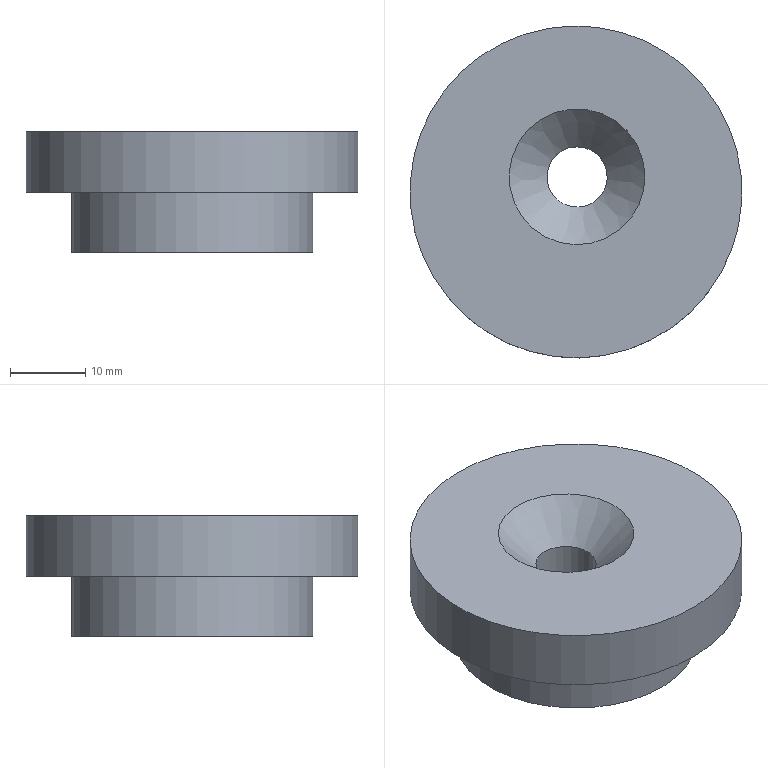Component | NX | PUNCHING_DIE | 1 solid | 7 faces | box 44 x 44 x 16 mm | volume 17349 mm3 | plane 3 | cylinder 3 | cone 1 | commonest cylinder face diameters 44 x1 32 x1 8 x1
STEP:
#1=CARTESIAN_POINT('',(0.,0.,0.));
#2=DIRECTION('',(0.,0.,1.));
#3=DIRECTION('',(1.,0.,0.));
#4=AXIS2_PLACEMENT_3D('',#1,#2,#3);
#5=CARTESIAN_POINT('',(11.337,1.54,-38.5));
#6=VERTEX_POINT('',#5);
#7=CARTESIAN_POINT('',(3.947,-1.525,-38.5));
#8=VERTEX_POINT('',#7);
#9=CARTESIAN_POINT('',(7.642,0.007455,-38.5));
#10=DIRECTION('',(0.,0.,-1.));
#11=DIRECTION('',(0.9237,0.383,0.));
#12=AXIS2_PLACEMENT_3D('',#9,#10,#11);
#13=CIRCLE('',#12,4.);
#14=CARTESIAN_POINT('',(1.371,12.78,-38.5));
#15=DIRECTION('',(0.,0.,-1.));
#16=DIRECTION('',(0.9237,0.383,0.));
#17=AXIS2_PLACEMENT_3D('',#14,#15,#16);
#18=PLANE('',#17);
#19=CARTESIAN_POINT('',(0.9,14.2));
#20=DIRECTION('',(1.,0.));
#21=AXIS2_PLACEMENT_2D('',#19,#20);
#22=CIRCLE('',#21,4.);
#23=(GEOMETRIC_REPRESENTATION_CONTEXT(2)PARAMETRIC_REPRESENTATION_CONTEXT()REPRESENTATION_CONTEXT('',''));
#24=DEFINITIONAL_REPRESENTATION('',(#22),#23);
#25=PCURVE('',#18,#24);
#26=CARTESIAN_POINT('',(7.642,0.007455,-80.5));
#27=DIRECTION('',(0.,0.,1.));
#28=DIRECTION('',(-0.9237,-0.383,0.));
#29=AXIS2_PLACEMENT_3D('',#26,#27,#28);
#30=CYLINDRICAL_SURFACE('',#29,4.);
#31=CARTESIAN_POINT('',(3.142,42.));
#32=DIRECTION('',(-1.,0.));
#33=VECTOR('',#32,1.);
#34=LINE('',#31,#33);
#35=(GEOMETRIC_REPRESENTATION_CONTEXT(2)PARAMETRIC_REPRESENTATION_CONTEXT()REPRESENTATION_CONTEXT('',''));
#36=DEFINITIONAL_REPRESENTATION('',(#34),#35);
#37=PCURVE('',#30,#36);
#38=SURFACE_CURVE('',#13,(#25,#37),.PCURVE_S1.);
#39=EDGE_CURVE('',#6,#8,#38,.T.);
#40=ORIENTED_EDGE('',*,*,#39,.F.);
#41=CARTESIAN_POINT('',(7.642,0.007455,-38.5));
#42=DIRECTION('',(0.,0.,-1.));
#43=DIRECTION('',(0.9237,0.383,0.));
#44=AXIS2_PLACEMENT_3D('',#41,#42,#43);
#45=CIRCLE('',#44,4.);
#46=CARTESIAN_POINT('',(0.9,14.2));
#47=DIRECTION('',(1.,0.));
#48=AXIS2_PLACEMENT_2D('',#46,#47);
#49=CIRCLE('',#48,4.);
#50=(GEOMETRIC_REPRESENTATION_CONTEXT(2)PARAMETRIC_REPRESENTATION_CONTEXT()REPRESENTATION_CONTEXT('',''));
#51=DEFINITIONAL_REPRESENTATION('',(#49),#50);
#52=PCURVE('',#18,#51);
#53=CARTESIAN_POINT('',(9.425,42.));
#54=DIRECTION('',(-1.,0.));
#55=VECTOR('',#54,1.);
#56=LINE('',#53,#55);
#57=(GEOMETRIC_REPRESENTATION_CONTEXT(2)PARAMETRIC_REPRESENTATION_CONTEXT()REPRESENTATION_CONTEXT('',''));
#58=DEFINITIONAL_REPRESENTATION('',(#56),#57);
#59=PCURVE('',#30,#58);
#60=SURFACE_CURVE('',#45,(#52,#59),.PCURVE_S1.);
#61=EDGE_CURVE('',#8,#6,#60,.T.);
#62=ORIENTED_EDGE('',*,*,#61,.F.);
#63=EDGE_LOOP('',(#40,#62));
#64=FACE_BOUND('',#63,.T.);
#65=CARTESIAN_POINT('',(-7.28,-8.129,-38.5));
#66=VERTEX_POINT('',#65);
#67=CARTESIAN_POINT('',(7.5,-2.,-38.5));
#68=DIRECTION('',(0.,0.,1.));
#69=DIRECTION('',(-0.9237,-0.383,0.));
#70=AXIS2_PLACEMENT_3D('',#67,#68,#69);
#71=CIRCLE('',#70,16.);
#72=CARTESIAN_POINT('',(-16.,16.));
#73=CARTESIAN_POINT('',(-16.,43.713));
#74=CARTESIAN_POINT('',(8.,29.856));
#75=CARTESIAN_POINT('',(32.,16.));
#76=CARTESIAN_POINT('',(8.,2.144));
#77=CARTESIAN_POINT('',(-16.,-11.713));
#78=CARTESIAN_POINT('',(-16.,16.));
#79=(BOUNDED_CURVE()B_SPLINE_CURVE(2,(#72,#73,#74,#75,#76,#77,#78),.UNSPECIFIED.,.T.,.F.)B_SPLINE_CURVE_WITH_KNOTS((1,2,2,2,2,1),(-2.094,0.,2.094,4.189,6.283,8.378),.UNSPECIFIED.)CURVE()GEOMETRIC_REPRESENTATION_ITEM()RATIONAL_B_SPLINE_CURVE((1.,0.5,1.,0.5,1.,0.5,1.))REPRESENTATION_ITEM(''));
#80=(GEOMETRIC_REPRESENTATION_CONTEXT(2)PARAMETRIC_REPRESENTATION_CONTEXT()REPRESENTATION_CONTEXT('',''));
#81=DEFINITIONAL_REPRESENTATION('',(#79),#80);
#82=PCURVE('',#18,#81);
#83=CARTESIAN_POINT('',(7.5,-2.,-22.5));
#84=DIRECTION('',(0.,0.,1.));
#85=DIRECTION('',(-0.9237,-0.383,0.));
#86=AXIS2_PLACEMENT_3D('',#83,#84,#85);
#87=CYLINDRICAL_SURFACE('',#86,16.);
#88=CARTESIAN_POINT('',(0.,-16.));
#89=DIRECTION('',(1.,0.));
#90=VECTOR('',#89,1.);
#91=LINE('',#88,#90);
#92=(GEOMETRIC_REPRESENTATION_CONTEXT(2)PARAMETRIC_REPRESENTATION_CONTEXT()REPRESENTATION_CONTEXT('',''));
#93=DEFINITIONAL_REPRESENTATION('',(#91),#92);
#94=PCURVE('',#87,#93);
#95=SURFACE_CURVE('',#71,(#82,#94),.PCURVE_S1.);
#96=EDGE_CURVE('',#66,#66,#95,.T.);
#97=ORIENTED_EDGE('',*,*,#96,.F.);
#98=EDGE_LOOP('',(#97));
#99=FACE_BOUND('',#98,.T.);
#100=ADVANCED_FACE('',(#64,#99),#18,.T.);
#101=CARTESIAN_POINT('',(-0.6717,-3.44,-22.5));
#102=VERTEX_POINT('',#101);
#103=CARTESIAN_POINT('',(7.642,0.007455,-22.5));
#104=DIRECTION('',(0.,0.,-1.));
#105=DIRECTION('',(-0.9237,-0.383,0.));
#106=AXIS2_PLACEMENT_3D('',#103,#104,#105);
#107=CIRCLE('',#106,9.);
#108=CARTESIAN_POINT('',(4.819,4.466,-22.5));
#109=DIRECTION('',(0.,0.,1.));
#110=DIRECTION('',(-0.9237,-0.383,0.));
#111=AXIS2_PLACEMENT_3D('',#108,#109,#110);
#112=PLANE('',#111);
#113=CARTESIAN_POINT('',(8.1,5.2));
#114=CARTESIAN_POINT('',(8.1,-10.388));
#115=CARTESIAN_POINT('',(-5.4,-2.594));
#116=CARTESIAN_POINT('',(-18.9,5.2));
#117=CARTESIAN_POINT('',(-5.4,12.994));
#118=CARTESIAN_POINT('',(8.1,20.788));
#119=CARTESIAN_POINT('',(8.1,5.2));
#120=(BOUNDED_CURVE()B_SPLINE_CURVE(2,(#113,#114,#115,#116,#117,#118,#119),.UNSPECIFIED.,.T.,.F.)B_SPLINE_CURVE_WITH_KNOTS((1,2,2,2,2,1),(-2.094,0.,2.094,4.189,6.283,8.378),.UNSPECIFIED.)CURVE()GEOMETRIC_REPRESENTATION_ITEM()RATIONAL_B_SPLINE_CURVE((1.,0.5,1.,0.5,1.,0.5,1.))REPRESENTATION_ITEM(''));
#121=(GEOMETRIC_REPRESENTATION_CONTEXT(2)PARAMETRIC_REPRESENTATION_CONTEXT()REPRESENTATION_CONTEXT('',''));
#122=DEFINITIONAL_REPRESENTATION('',(#120),#121);
#123=PCURVE('',#112,#122);
#124=CARTESIAN_POINT('',(7.642,0.007455,-27.5));
#125=DIRECTION('',(0.,0.,1.));
#126=DIRECTION('',(-0.9237,-0.383,0.));
#127=AXIS2_PLACEMENT_3D('',#124,#125,#126);
#128=CONICAL_SURFACE('',#127,4.,0.7854);
#129=CARTESIAN_POINT('',(6.283,5.));
#130=DIRECTION('',(-1.,0.));
#131=VECTOR('',#130,1.);
#132=LINE('',#129,#131);
#133=(GEOMETRIC_REPRESENTATION_CONTEXT(2)PARAMETRIC_REPRESENTATION_CONTEXT()REPRESENTATION_CONTEXT('',''));
#134=DEFINITIONAL_REPRESENTATION('',(#132),#133);
#135=PCURVE('',#128,#134);
#136=SURFACE_CURVE('',#107,(#123,#135),.PCURVE_S1.);
#137=EDGE_CURVE('',#102,#102,#136,.T.);
#138=ORIENTED_EDGE('',*,*,#137,.T.);
#139=EDGE_LOOP('',(#138));
#140=FACE_BOUND('',#139,.T.);
#141=CARTESIAN_POINT('',(-12.822,-10.427,-22.5));
#142=VERTEX_POINT('',#141);
#143=CARTESIAN_POINT('',(7.5,-2.,-22.5));
#144=DIRECTION('',(0.,0.,1.));
#145=DIRECTION('',(-0.9237,-0.383,0.));
#146=AXIS2_PLACEMENT_3D('',#143,#144,#145);
#147=CIRCLE('',#146,22.);
#148=CARTESIAN_POINT('',(0.,7.));
#149=DIRECTION('',(1.,0.));
#150=AXIS2_PLACEMENT_2D('',#148,#149);
#151=CIRCLE('',#150,22.);
#152=(GEOMETRIC_REPRESENTATION_CONTEXT(2)PARAMETRIC_REPRESENTATION_CONTEXT()REPRESENTATION_CONTEXT('',''));
#153=DEFINITIONAL_REPRESENTATION('',(#151),#152);
#154=PCURVE('',#112,#153);
#155=CARTESIAN_POINT('',(7.5,-2.,-22.5));
#156=DIRECTION('',(0.,0.,1.));
#157=DIRECTION('',(-0.9237,-0.383,0.));
#158=AXIS2_PLACEMENT_3D('',#155,#156,#157);
#159=CYLINDRICAL_SURFACE('',#158,22.);
#160=CARTESIAN_POINT('',(0.,0.));
#161=DIRECTION('',(1.,0.));
#162=VECTOR('',#161,1.);
#163=LINE('',#160,#162);
#164=(GEOMETRIC_REPRESENTATION_CONTEXT(2)PARAMETRIC_REPRESENTATION_CONTEXT()REPRESENTATION_CONTEXT('',''));
#165=DEFINITIONAL_REPRESENTATION('',(#163),#164);
#166=PCURVE('',#159,#165);
#167=SURFACE_CURVE('',#147,(#154,#166),.PCURVE_S1.);
#168=EDGE_CURVE('',#142,#142,#167,.T.);
#169=ORIENTED_EDGE('',*,*,#168,.T.);
#170=EDGE_LOOP('',(#169));
#171=FACE_BOUND('',#170,.T.);
#172=ADVANCED_FACE('',(#140,#171),#112,.T.);
#173=CARTESIAN_POINT('',(-12.822,-10.427,-30.5));
#174=VERTEX_POINT('',#173);
#175=CARTESIAN_POINT('',(7.5,-2.,-30.5));
#176=DIRECTION('',(0.,0.,1.));
#177=DIRECTION('',(-0.9237,-0.383,0.));
#178=AXIS2_PLACEMENT_3D('',#175,#176,#177);
#179=CIRCLE('',#178,22.);
#180=CARTESIAN_POINT('',(0.,-8.));
#181=DIRECTION('',(1.,0.));
#182=VECTOR('',#181,1.);
#183=LINE('',#180,#182);
#184=(GEOMETRIC_REPRESENTATION_CONTEXT(2)PARAMETRIC_REPRESENTATION_CONTEXT()REPRESENTATION_CONTEXT('',''));
#185=DEFINITIONAL_REPRESENTATION('',(#183),#184);
#186=PCURVE('',#159,#185);
#187=CARTESIAN_POINT('',(-0.9271,18.322,-30.5));
#188=DIRECTION('',(0.,0.,-1.));
#189=DIRECTION('',(0.9237,0.383,0.));
#190=AXIS2_PLACEMENT_3D('',#187,#188,#189);
#191=PLANE('',#190);
#192=CARTESIAN_POINT('',(-22.,22.));
#193=CARTESIAN_POINT('',(-22.,60.105));
#194=CARTESIAN_POINT('',(11.,41.053));
#195=CARTESIAN_POINT('',(44.,22.));
#196=CARTESIAN_POINT('',(11.,2.947));
#197=CARTESIAN_POINT('',(-22.,-16.105));
#198=CARTESIAN_POINT('',(-22.,22.));
#199=(BOUNDED_CURVE()B_SPLINE_CURVE(2,(#192,#193,#194,#195,#196,#197,#198),.UNSPECIFIED.,.T.,.F.)B_SPLINE_CURVE_WITH_KNOTS((1,2,2,2,2,1),(-2.094,0.,2.094,4.189,6.283,8.378),.UNSPECIFIED.)CURVE()GEOMETRIC_REPRESENTATION_ITEM()RATIONAL_B_SPLINE_CURVE((1.,0.5,1.,0.5,1.,0.5,1.))REPRESENTATION_ITEM(''));
#200=(GEOMETRIC_REPRESENTATION_CONTEXT(2)PARAMETRIC_REPRESENTATION_CONTEXT()REPRESENTATION_CONTEXT('',''));
#201=DEFINITIONAL_REPRESENTATION('',(#199),#200);
#202=PCURVE('',#191,#201);
#203=SURFACE_CURVE('',#179,(#186,#202),.PCURVE_S1.);
#204=EDGE_CURVE('',#174,#174,#203,.T.);
#205=ORIENTED_EDGE('',*,*,#204,.T.);
#206=CARTESIAN_POINT('',(-12.822,-10.427,-30.5));
#207=CARTESIAN_POINT('',(-12.822,-10.427,-22.5));
#208=B_SPLINE_CURVE_WITH_KNOTS('',1,(#206,#207),.UNSPECIFIED.,.F.,.F.,(2,2),(-8.,0.),.PIECEWISE_BEZIER_KNOTS.);
#209=CARTESIAN_POINT('',(6.283,0.));
#210=DIRECTION('',(0.,1.));
#211=VECTOR('',#210,1.);
#212=LINE('',#209,#211);
#213=(GEOMETRIC_REPRESENTATION_CONTEXT(2)PARAMETRIC_REPRESENTATION_CONTEXT()REPRESENTATION_CONTEXT('',''));
#214=DEFINITIONAL_REPRESENTATION('',(#212),#213);
#215=PCURVE('',#159,#214);
#216=CARTESIAN_POINT('',(0.,0.));
#217=DIRECTION('',(0.,1.));
#218=VECTOR('',#217,1.);
#219=LINE('',#216,#218);
#220=(GEOMETRIC_REPRESENTATION_CONTEXT(2)PARAMETRIC_REPRESENTATION_CONTEXT()REPRESENTATION_CONTEXT('',''));
#221=DEFINITIONAL_REPRESENTATION('',(#219),#220);
#222=PCURVE('',#159,#221);
#223=SEAM_CURVE('',#208,(#215,#222),.PCURVE_S1.);
#224=EDGE_CURVE('',#174,#142,#223,.T.);
#225=ORIENTED_EDGE('',*,*,#224,.T.);
#226=ORIENTED_EDGE('',*,*,#168,.F.);
#227=ORIENTED_EDGE('',*,*,#224,.F.);
#228=EDGE_LOOP('',(#205,#225,#226,#227));
#229=FACE_BOUND('',#228,.T.);
#230=ADVANCED_FACE('',(#229),#159,.T.);
#231=CARTESIAN_POINT('',(-7.28,-8.129,-30.5));
#232=VERTEX_POINT('',#231);
#233=CARTESIAN_POINT('',(7.5,-2.,-30.5));
#234=DIRECTION('',(0.,0.,1.));
#235=DIRECTION('',(-0.9237,-0.383,0.));
#236=AXIS2_PLACEMENT_3D('',#233,#234,#235);
#237=CIRCLE('',#236,16.);
#238=CARTESIAN_POINT('',(-16.,22.));
#239=CARTESIAN_POINT('',(-16.,49.713));
#240=CARTESIAN_POINT('',(8.,35.856));
#241=CARTESIAN_POINT('',(32.,22.));
#242=CARTESIAN_POINT('',(8.,8.144));
#243=CARTESIAN_POINT('',(-16.,-5.713));
#244=CARTESIAN_POINT('',(-16.,22.));
#245=(BOUNDED_CURVE()B_SPLINE_CURVE(2,(#238,#239,#240,#241,#242,#243,#244),.UNSPECIFIED.,.T.,.F.)B_SPLINE_CURVE_WITH_KNOTS((1,2,2,2,2,1),(-2.094,0.,2.094,4.189,6.283,8.378),.UNSPECIFIED.)CURVE()GEOMETRIC_REPRESENTATION_ITEM()RATIONAL_B_SPLINE_CURVE((1.,0.5,1.,0.5,1.,0.5,1.))REPRESENTATION_ITEM(''));
#246=(GEOMETRIC_REPRESENTATION_CONTEXT(2)PARAMETRIC_REPRESENTATION_CONTEXT()REPRESENTATION_CONTEXT('',''));
#247=DEFINITIONAL_REPRESENTATION('',(#245),#246);
#248=PCURVE('',#191,#247);
#249=CARTESIAN_POINT('',(0.,-8.));
#250=DIRECTION('',(1.,0.));
#251=VECTOR('',#250,1.);
#252=LINE('',#249,#251);
#253=(GEOMETRIC_REPRESENTATION_CONTEXT(2)PARAMETRIC_REPRESENTATION_CONTEXT()REPRESENTATION_CONTEXT('',''));
#254=DEFINITIONAL_REPRESENTATION('',(#252),#253);
#255=PCURVE('',#87,#254);
#256=SURFACE_CURVE('',#237,(#248,#255),.PCURVE_S1.);
#257=EDGE_CURVE('',#232,#232,#256,.T.);
#258=ORIENTED_EDGE('',*,*,#257,.T.);
#259=EDGE_LOOP('',(#258));
#260=FACE_BOUND('',#259,.T.);
#261=ORIENTED_EDGE('',*,*,#204,.F.);
#262=EDGE_LOOP('',(#261));
#263=FACE_BOUND('',#262,.T.);
#264=ADVANCED_FACE('',(#260,#263),#191,.T.);
#265=ORIENTED_EDGE('',*,*,#96,.T.);
#266=CARTESIAN_POINT('',(-7.28,-8.129,-38.5));
#267=CARTESIAN_POINT('',(-7.28,-8.129,-30.5));
#268=B_SPLINE_CURVE_WITH_KNOTS('',1,(#266,#267),.UNSPECIFIED.,.F.,.F.,(2,2),(-16.,-8.),.PIECEWISE_BEZIER_KNOTS.);
#269=CARTESIAN_POINT('',(6.283,0.));
#270=DIRECTION('',(0.,1.));
#271=VECTOR('',#270,1.);
#272=LINE('',#269,#271);
#273=(GEOMETRIC_REPRESENTATION_CONTEXT(2)PARAMETRIC_REPRESENTATION_CONTEXT()REPRESENTATION_CONTEXT('',''));
#274=DEFINITIONAL_REPRESENTATION('',(#272),#273);
#275=PCURVE('',#87,#274);
#276=CARTESIAN_POINT('',(0.,0.));
#277=DIRECTION('',(0.,1.));
#278=VECTOR('',#277,1.);
#279=LINE('',#276,#278);
#280=(GEOMETRIC_REPRESENTATION_CONTEXT(2)PARAMETRIC_REPRESENTATION_CONTEXT()REPRESENTATION_CONTEXT('',''));
#281=DEFINITIONAL_REPRESENTATION('',(#279),#280);
#282=PCURVE('',#87,#281);
#283=SEAM_CURVE('',#268,(#275,#282),.PCURVE_S1.);
#284=EDGE_CURVE('',#66,#232,#283,.T.);
#285=ORIENTED_EDGE('',*,*,#284,.T.);
#286=ORIENTED_EDGE('',*,*,#257,.F.);
#287=ORIENTED_EDGE('',*,*,#284,.F.);
#288=EDGE_LOOP('',(#265,#285,#286,#287));
#289=FACE_BOUND('',#288,.T.);
#290=ADVANCED_FACE('',(#289),#87,.T.);
#291=CARTESIAN_POINT('',(3.947,-1.525,-27.5));
#292=VERTEX_POINT('',#291);
#293=CARTESIAN_POINT('',(7.642,0.007455,-27.5));
#294=DIRECTION('',(0.,0.,1.));
#295=DIRECTION('',(-0.9237,-0.383,0.));
#296=AXIS2_PLACEMENT_3D('',#293,#294,#295);
#297=CIRCLE('',#296,4.);
#298=CARTESIAN_POINT('',(0.,53.));
#299=DIRECTION('',(1.,0.));
#300=VECTOR('',#299,1.);
#301=LINE('',#298,#300);
#302=(GEOMETRIC_REPRESENTATION_CONTEXT(2)PARAMETRIC_REPRESENTATION_CONTEXT()REPRESENTATION_CONTEXT('',''));
#303=DEFINITIONAL_REPRESENTATION('',(#301),#302);
#304=PCURVE('',#30,#303);
#305=CARTESIAN_POINT('',(0.,0.));
#306=DIRECTION('',(1.,0.));
#307=VECTOR('',#306,1.);
#308=LINE('',#305,#307);
#309=(GEOMETRIC_REPRESENTATION_CONTEXT(2)PARAMETRIC_REPRESENTATION_CONTEXT()REPRESENTATION_CONTEXT('',''));
#310=DEFINITIONAL_REPRESENTATION('',(#308),#309);
#311=PCURVE('',#128,#310);
#312=SURFACE_CURVE('',#297,(#304,#311),.PCURVE_S1.);
#313=EDGE_CURVE('',#292,#292,#312,.T.);
#314=ORIENTED_EDGE('',*,*,#313,.F.);
#315=CARTESIAN_POINT('',(3.947,-1.525,-38.5));
#316=CARTESIAN_POINT('',(3.947,-1.525,-27.5));
#317=B_SPLINE_CURVE_WITH_KNOTS('',1,(#315,#316),.UNSPECIFIED.,.F.,.F.,(2,2),(42.,53.),.PIECEWISE_BEZIER_KNOTS.);
#318=CARTESIAN_POINT('',(0.,0.));
#319=DIRECTION('',(0.,1.));
#320=VECTOR('',#319,1.);
#321=LINE('',#318,#320);
#322=(GEOMETRIC_REPRESENTATION_CONTEXT(2)PARAMETRIC_REPRESENTATION_CONTEXT()REPRESENTATION_CONTEXT('',''));
#323=DEFINITIONAL_REPRESENTATION('',(#321),#322);
#324=PCURVE('',#30,#323);
#325=CARTESIAN_POINT('',(6.283,0.));
#326=DIRECTION('',(0.,1.));
#327=VECTOR('',#326,1.);
#328=LINE('',#325,#327);
#329=(GEOMETRIC_REPRESENTATION_CONTEXT(2)PARAMETRIC_REPRESENTATION_CONTEXT()REPRESENTATION_CONTEXT('',''));
#330=DEFINITIONAL_REPRESENTATION('',(#328),#329);
#331=PCURVE('',#30,#330);
#332=SEAM_CURVE('',#317,(#324,#331),.PCURVE_S1.);
#333=EDGE_CURVE('',#8,#292,#332,.T.);
#334=ORIENTED_EDGE('',*,*,#333,.F.);
#335=ORIENTED_EDGE('',*,*,#39,.F.);
#336=ORIENTED_EDGE('',*,*,#61,.F.);
#337=ORIENTED_EDGE('',*,*,#333,.T.);
#338=EDGE_LOOP('',(#314,#334,#335,#336,#337));
#339=FACE_BOUND('',#338,.F.);
#340=ADVANCED_FACE('',(#339),#30,.F.);
#341=ORIENTED_EDGE('',*,*,#137,.T.);
#342=CARTESIAN_POINT('',(3.947,-1.525,-27.5));
#343=CARTESIAN_POINT('',(-0.6717,-3.44,-22.5));
#344=B_SPLINE_CURVE_WITH_KNOTS('',1,(#342,#343),.UNSPECIFIED.,.F.,.F.,(2,2),(0.,7.071),.PIECEWISE_BEZIER_KNOTS.);
#345=CARTESIAN_POINT('',(0.,0.));
#346=DIRECTION('',(0.,1.));
#347=VECTOR('',#346,1.);
#348=LINE('',#345,#347);
#349=(GEOMETRIC_REPRESENTATION_CONTEXT(2)PARAMETRIC_REPRESENTATION_CONTEXT()REPRESENTATION_CONTEXT('',''));
#350=DEFINITIONAL_REPRESENTATION('',(#348),#349);
#351=PCURVE('',#128,#350);
#352=CARTESIAN_POINT('',(6.283,0.));
#353=DIRECTION('',(0.,1.));
#354=VECTOR('',#353,1.);
#355=LINE('',#352,#354);
#356=(GEOMETRIC_REPRESENTATION_CONTEXT(2)PARAMETRIC_REPRESENTATION_CONTEXT()REPRESENTATION_CONTEXT('',''));
#357=DEFINITIONAL_REPRESENTATION('',(#355),#356);
#358=PCURVE('',#128,#357);
#359=SEAM_CURVE('',#344,(#351,#358),.PCURVE_S1.);
#360=EDGE_CURVE('',#292,#102,#359,.T.);
#361=ORIENTED_EDGE('',*,*,#360,.F.);
#362=ORIENTED_EDGE('',*,*,#313,.T.);
#363=ORIENTED_EDGE('',*,*,#360,.T.);
#364=EDGE_LOOP('',(#341,#361,#362,#363));
#365=FACE_BOUND('',#364,.F.);
#366=ADVANCED_FACE('',(#365),#128,.F.);
#367=CLOSED_SHELL('',(#100,#172,#230,#264,#290,#340,#366));
#368=MANIFOLD_SOLID_BREP('',#367);
#369=(LENGTH_UNIT()NAMED_UNIT(*)SI_UNIT(.MILLI.,.METRE.));
#370=UNCERTAINTY_MEASURE_WITH_UNIT(LENGTH_MEASURE(0.000005),#369,'','');
#371=(NAMED_UNIT(*)PLANE_ANGLE_UNIT()SI_UNIT($,.RADIAN.));
#372=(NAMED_UNIT(*)SI_UNIT($,.STERADIAN.)SOLID_ANGLE_UNIT());
#373=(GEOMETRIC_REPRESENTATION_CONTEXT(3)GLOBAL_UNCERTAINTY_ASSIGNED_CONTEXT((#370))GLOBAL_UNIT_ASSIGNED_CONTEXT((#369,#371,#372))REPRESENTATION_CONTEXT('',''));
#374=ADVANCED_BREP_SHAPE_REPRESENTATION('',(#4,#368),#373);